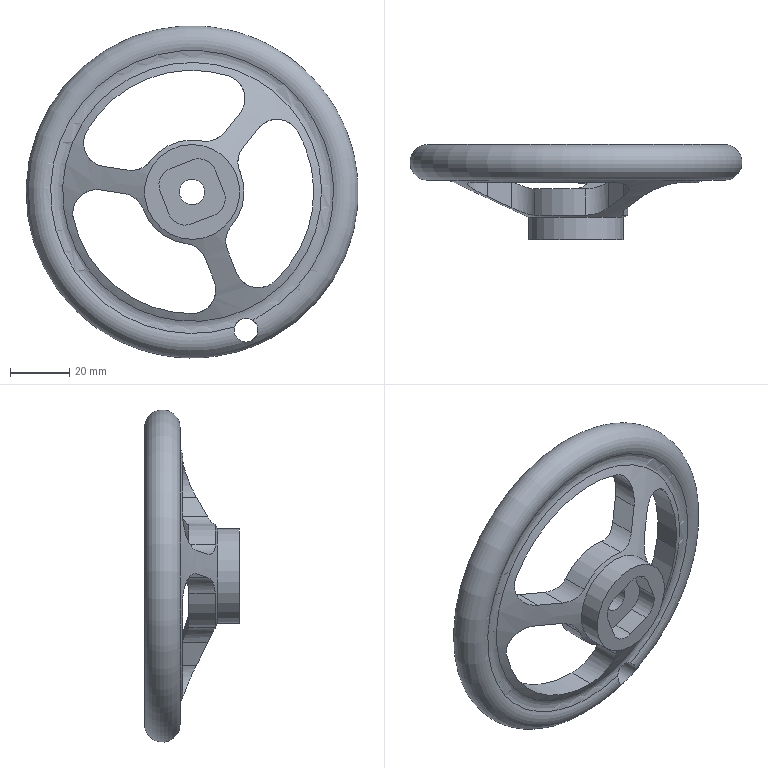Component | NX | HANDWHEEL | 1 solid | 46 faces | volume 61721 mm3 | cylinder 25 | plane 16 | torus 3 | cone 2 | commonest cylinder face diameters 16 x12 12 x4 35 x3 82 x3 32 x1 8.5 x1 8 x1